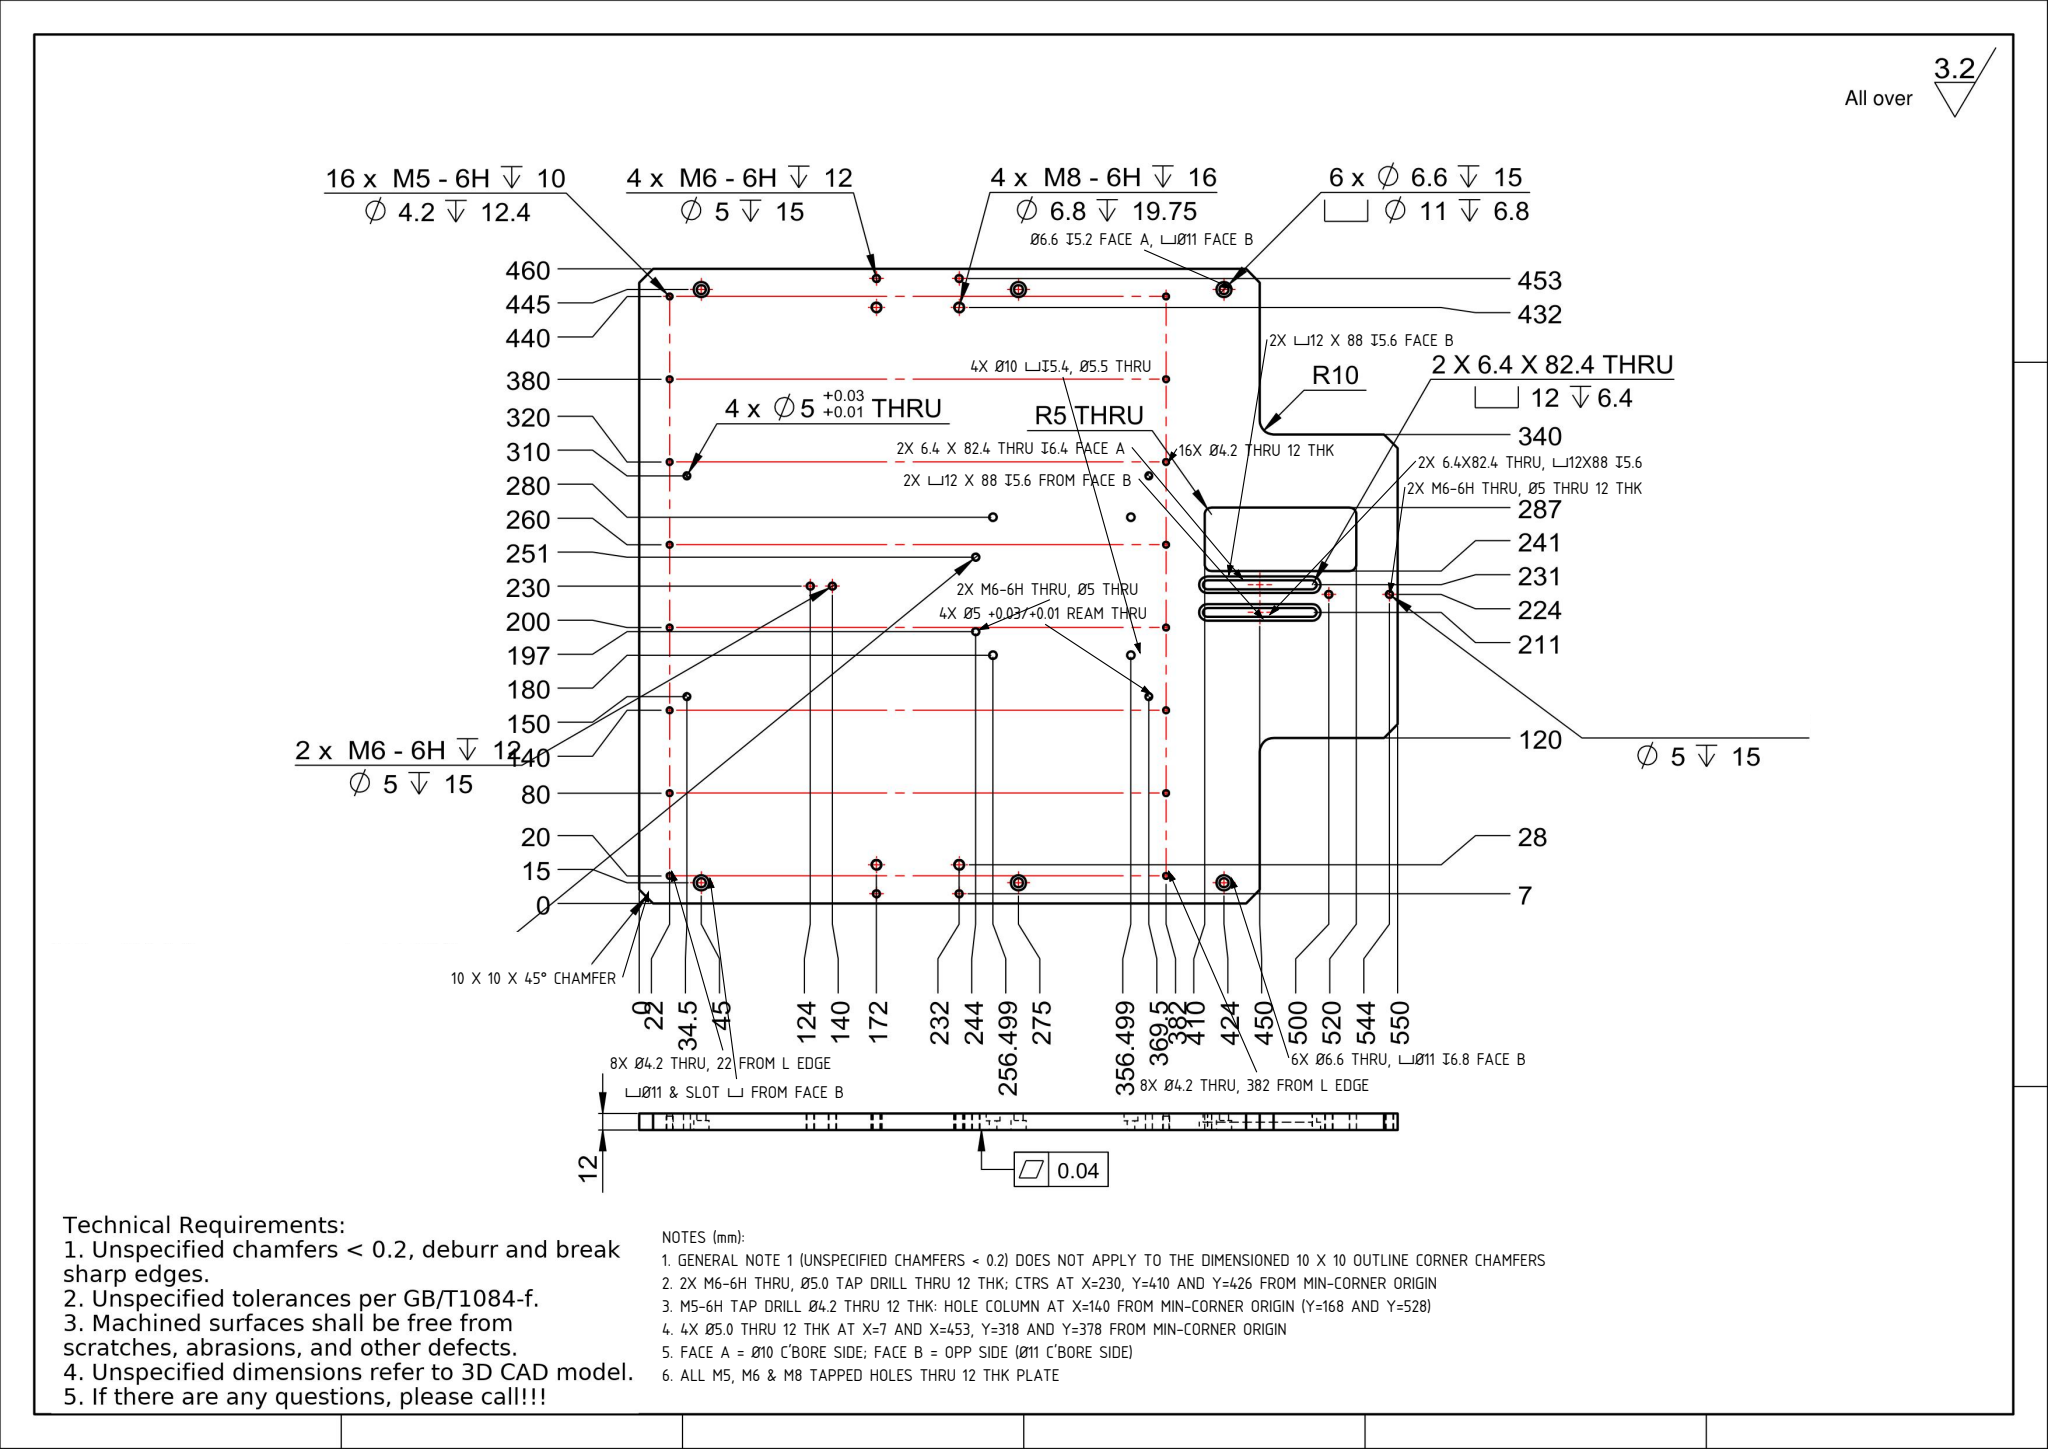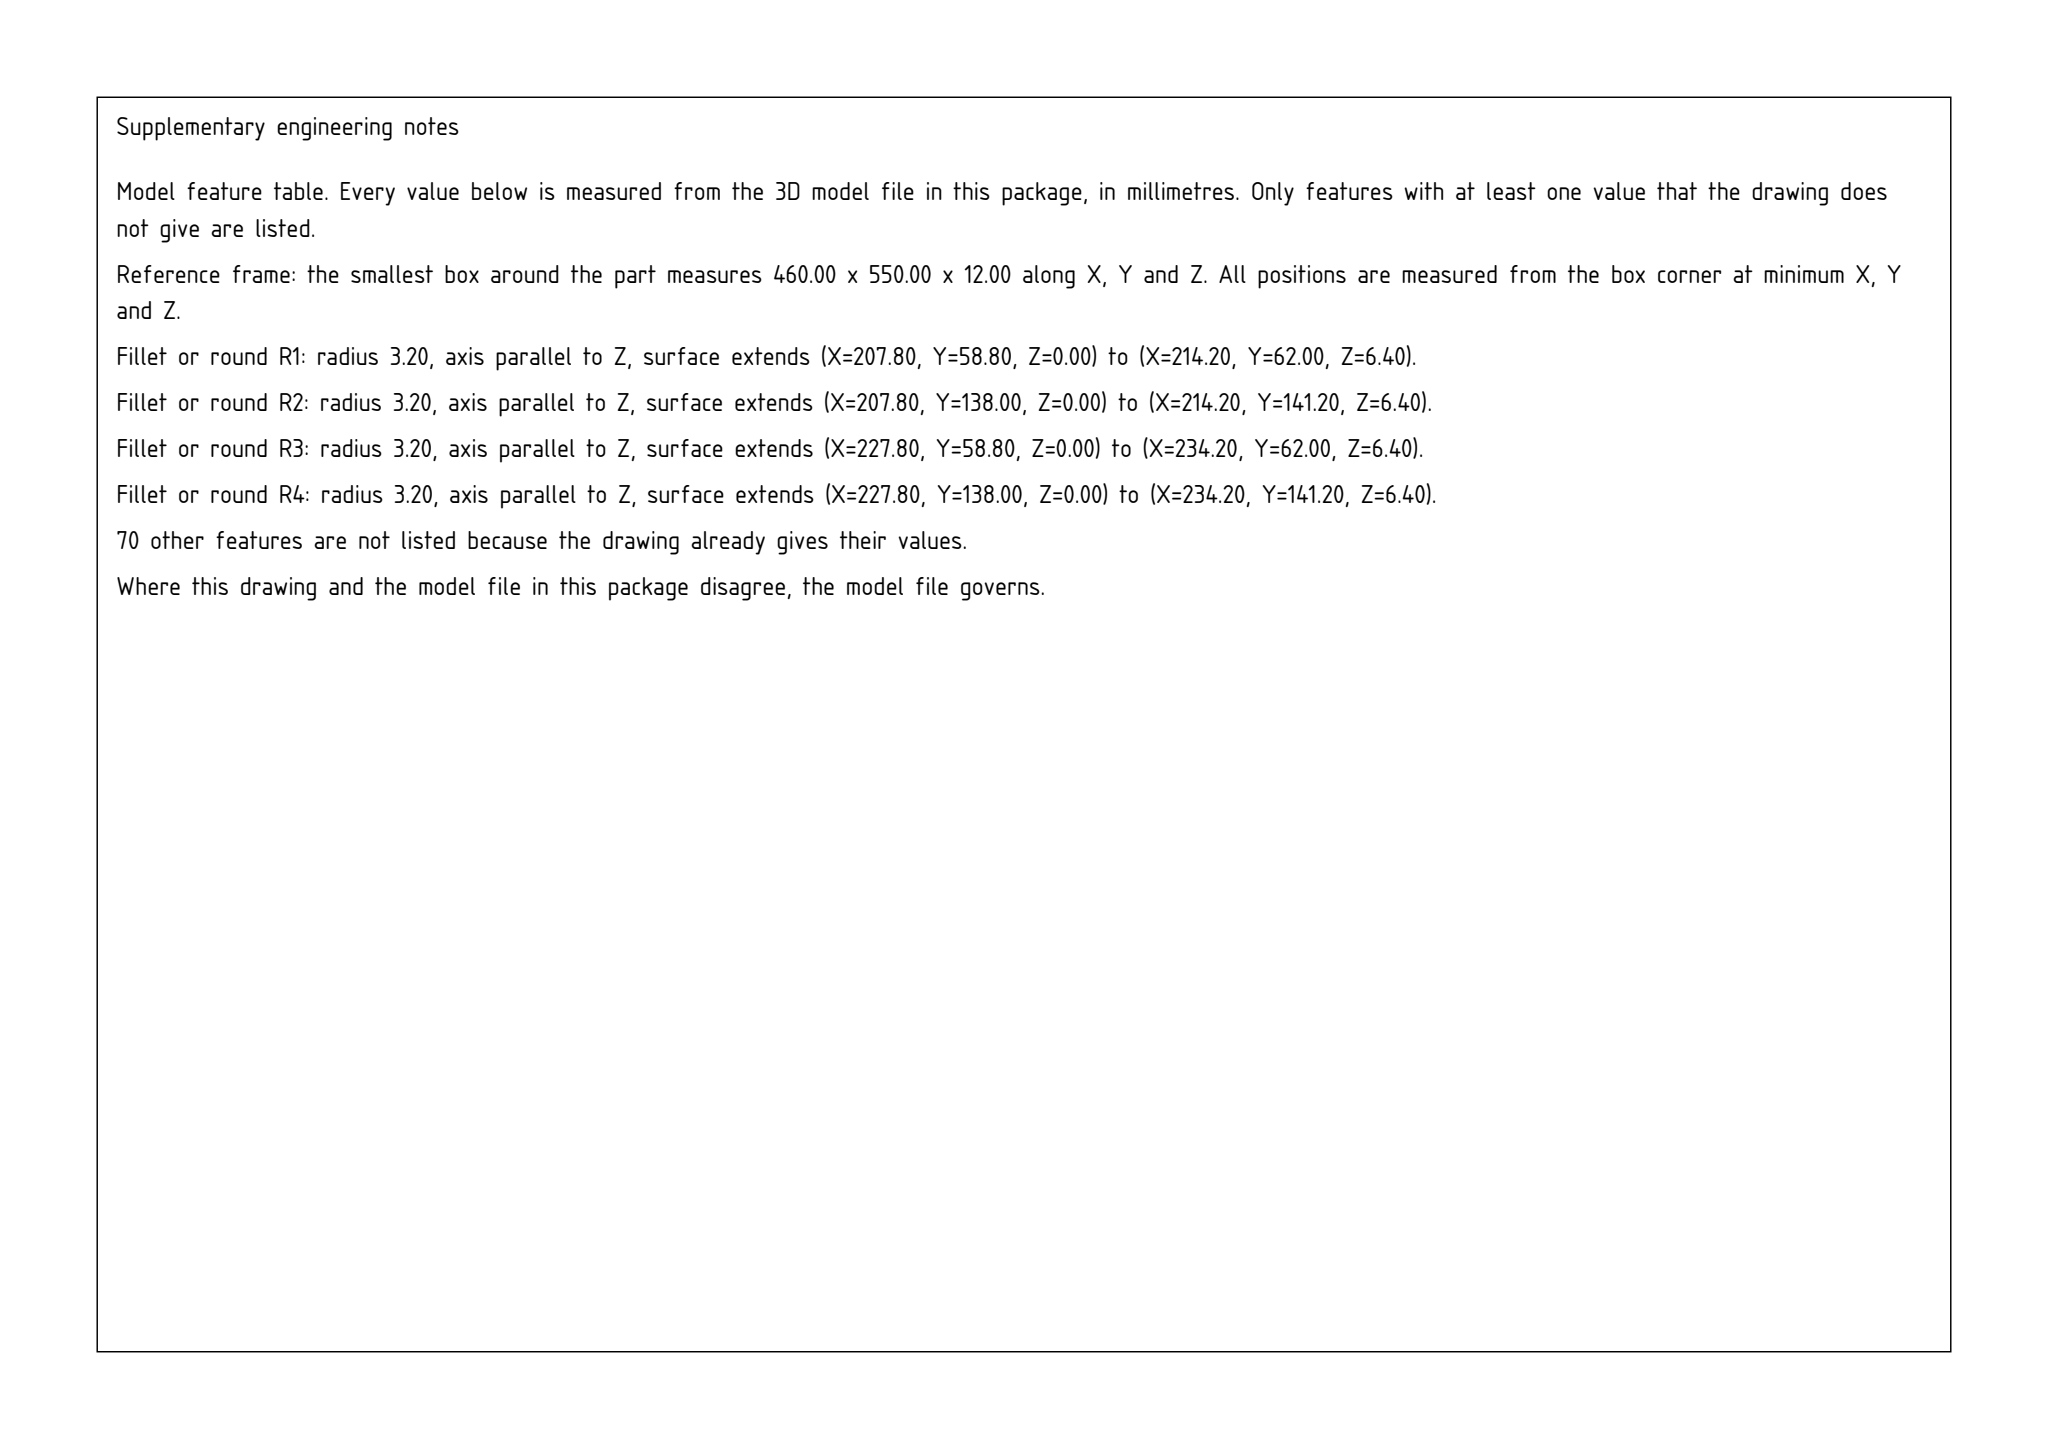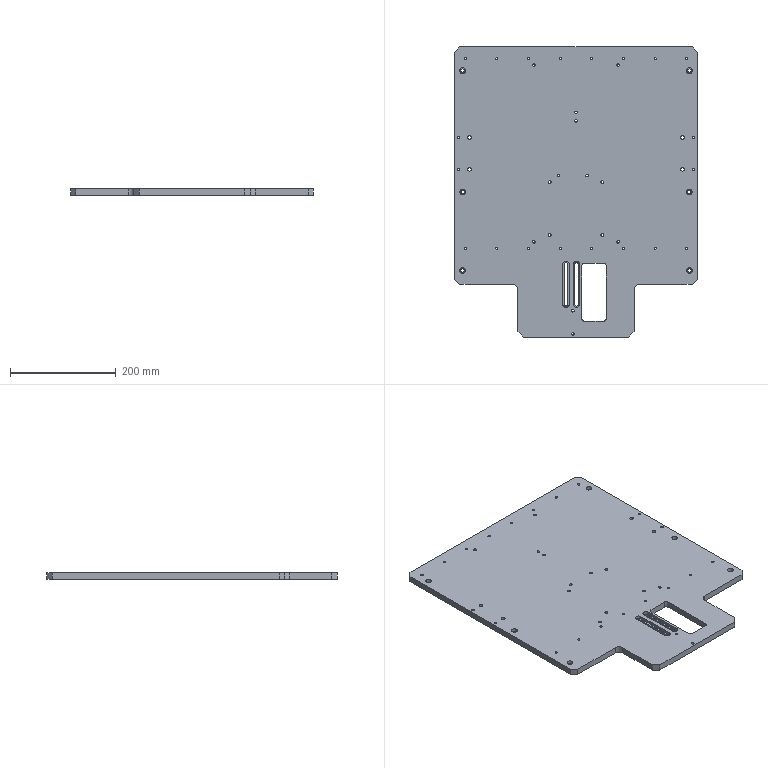Part | SolidWorks | mm | 1 solid | 162 faces | box 460 x 550 x 12 mm | volume 2651363 mm3 | cylinder 122 | plane 40 | commonest cylinder face diameters 4.2 x32 5 x28 10 x12 11 x12 6.6 x12 5.5 x8 6.8 x8 12 x4
Drawing notes:
SLOT C'BORE: 2X C'BORE 12 WIDE X 88 LG (R6 ENDS, END R CTRS AT 412 & 488 FROM LEFT EDGE), DP 5.6 FROM FACE B (OPPOSITE FACE TO THE Ø10 C'BORES), CL AT 211 & 231 FROM BOTTOM EDGE | from the solid: Ø12 slot-end arcs at (211,62),(211,138),(231,62),(231,138) run z 6.4→12 (depth 5.6 from the z=12 face, opposite the Ø10 c'bores at z 0→5.4); the z=6.4 c'bore floor planes extend y 56–144 x 12 wide (205–217 and 225–237), i.e. 88 long with R6 centers at y 62 & 138 = 488 & 412 from left edge (550-y).
SLOT THRU PORTION: 2X 6.4 WIDE X 82.4 LG SLOT (R3.2 ENDS), DP 6.4 FROM FACE A (Ø10 C'BORE FACE), CL AT 211 & 231 FROM BOTTOM EDGE | from the solid: Ø6.4 arcs z 0→6.4 at (211,62/138) & (231,62/138); planes x207.8/214.2 and x227.8/234.2, z 0–6.4
FACE DESIGNATION: 6X Ø6.6 DRILLED FROM FACE A DP 5.2; Ø11 C'BORE DP 6.8 MACHINED FROM FACE B (OPPOSITE FACE); THE 4X Ø10 DP 5.4 C'BORES ARE FROM FACE A | from the solid: Ø6.6 z 0→5.2 and Ø11 z 5.2→12; Ø10 z 0→5.4 with Ø5.5 z 5.4→12
16X Ø4.2 TAP DRILL IS THRU THE FULL 12 THK PLATE (DRILL DP 12.4 CALLOUT = THRU) | from the solid: Ø4.2 holes z 0→12 at 20,80,140,200,260,320,380,440 on y=168 and y=528
10 X 10 X 45° CHAMFER (LEG 10 ON EACH EDGE) AT THE OUTLINE CORNERS, FULL 12 THK; INCL. CORNERS AT VERTICAL 0 / HORIZONTAL 450 AND VERTICAL 0 / HORIZONTAL 10 | from the solid: inclined_planes angle 45/45/90, size 10x10x12, bbox_from (0,100,0) and (0,540,0)
GENERAL NOTE 1 (UNSPECIFIED CHAMFERS < 0.2) DOES NOT APPLY TO THE DIMENSIONED 10 X 10 OUTLINE CORNER CHAMFERS | from the solid: inclined_planes 10x10x12 at 45° on outline corners
2X M6-6H THRU, Ø5.0 TAP DRILL THRU 12 THK; CTRS AT X=230, Y=410 AND Y=426 FROM MIN-CORNER ORIGIN | from the solid: cylinders: hole/bore dia 5.0, axis z, at [230.0,410.0] and [230.0,426.0], from 0.0 to 12.0 (full thickness)
M5-6H TAP DRILL Ø4.2 THRU 12 THK: HOLE COLUMN AT X=140 FROM MIN-CORNER ORIGIN (Y=168 AND Y=528) | from the solid: cylinders: hole/bore dia 4.2, axis z, at [140.0,168.0] and [140.0,528.0], from 0.0 to 12.0
4X Ø5 +0.03/+0.01 REAMED THRU 12 THK; CTRS AT X=150 AND X=310, Y=180.5 AND Y=515.5 FROM MIN-CORNER ORIGIN (180.5 = 369.5 FROM THE Y=550 EDGE) | from the solid: cylinders: hole/bore Ø5.0 axis z at (150,180.5), (310,180.5), (150,515.5), (310,515.5), from 0.0 to 12.0
M5-6H TAP DRILL Ø4.2 THRU 12 THK: HOLE ROW AT Y=168 FROM MIN-CORNER ORIGIN (382 FROM THE Y=550 EDGE); X=20, 80, 140, 200, 260, 320, 380, 440 | from the solid: cylinders: hole/bore Ø4.2 axis z at (20,168), (80,168), (140,168), (200,168), (260,168), (320,168), (380,168), (440,168), from 0.0 to 12.0
M5-6H TAP DRILL Ø4.2 THRU 12 THK: HOLE ROW AT Y=528 FROM MIN-CORNER ORIGIN (22 FROM THE Y=550 EDGE); X=20, 80, 140, 200, 260, 320, 380, 440 | from the solid: cylinders: hole/bore Ø4.2 axis z at y=528.0, x=20/80/140/200/260/320/380/440, from z=0.0 to z=12.0
2X M6-6H THRU, Ø5.0 TAP DRILL THRU FULL 12 THK; CTRS AT X=224, Y=6 AND Y=50 FROM MIN-CORNER ORIGIN | from the solid: cylinders: hole/bore dia 5.0, axis z at [224,6] and [224,50], from 0.0 to 12.0 (full plate THK)
2X M6-6H THRU, Ø5.0 TAP DRILL THRU FULL 12 THK; CTRS AT Y=306, X=197 AND X=251 FROM MIN-CORNER ORIGIN (REPLACES THE OVERLAPPED M6 CALLOUT) | from the solid: cylinders: hole/bore dia 5.0, axis z at [197,306] and [251,306], from 0.0 to 12.0
4X Ø5.0 THRU 12 THK AT X=7 AND X=453, Y=318 AND Y=378 FROM MIN-CORNER ORIGIN | from the solid: cylinders: hole/bore dia 5.0, axis z at [7,318], [7,378], [453,318], [453,378], from 0.0 to 12.0
FACE A = Ø10 C'BORE SIDE; FACE B = OPP SIDE (Ø11 C'BORE SIDE) | from the solid: Ø10 c'bores z=0->5.4 (Face A); Ø11 c'bores z=5.2->12.0 (Face B); plate z 0-12
6X Ø11 C'BORE & 2X SLOT C'BORE MACHINED FROM FACE B | from the solid: Ø11 bores from z=5.2 to 12; slot c'bore planes z=6.4 to 12 (x205-217 & x225-237, y56-144)
4X Ø10 CBORE DP 5.4 (Ø5.5 THRU) FROM FACE A | from the solid: Ø10 z=0->5.4 then Ø5.5 z=5.4->12 at (180/280, 193.5/293.5)
2X SLOT C'BORE: CBORE 12 WIDE X 88 LG DP 5.6 FROM FACE B | from the solid: slot c'bore floor plane z=6.4, top z=12 => 5.6 deep; width x205-217=12, y56-144=88
2X 6.4 X 82.4 THRU; CBORE 12 X 88 DP 5.6 FROM FACE B | from the solid: 6.4 wide slot z=0->6.4 breaks into 12 wide c'bore z=6.4->12; thru slot y62-138 + R3.2 ends = 82.4
ALL M5, M6 & M8 TAPPED HOLES THRU 12 THK PLATE | from the solid: Ø4.2, Ø5, Ø6.8 holes all from z=0.0 to z=12.0
6X Ø6.6 THRU, CBORE Ø11 DP 6.8 FROM FACE B | from the solid: Ø6.6 z=0->5.2 + Ø11 z=5.2->12 (6.8 deep) at x15/445, y126/275/505
build123d program:
from build123d import *

# Parameters (mm, degrees)
SKETCH1_W                                         = 460
SKETCH1_H                                         = 550
BOSS_EXTRUDE1_DEPTH                               = 12
SKETCH2_W                                         = 120
SKETCH2_H                                         = 100
CUT_EXTRUDE1_DEPTH                                = 12
FILLET1_R                                         = 10
CHAMFER1_SIZE                                     = 10
SKETCH3_W                                         = 46
SKETCH3_H                                         = 110
CUT_EXTRUDE2_DEPTH                                = 359.705
FILLET2_R                                         = 5
CUT_EXTRUDE3_DEPTH                                = 5.6
CUT_EXTRUDE4_DEPTH                                = 359.561
M6_TAPPED_HOLE1_D                                 = 5
M6_TAPPED_HOLE1_DEPTH                             = 15
M6_TAPPED_HOLE1_TIP                               = 1.502
LPATTERN1_COUNT                                   = 8
LPATTERN1_PITCH                                   = 60
LPATTERN1_COUNT_DIR2                              = 2
LPATTERN1_PITCH_DIR2                              = 360
M6_TAPPED_HOLE2_D                                 = 5
M6_TAPPED_HOLE2_DEPTH                             = 15
M6_TAPPED_HOLE2_TIP                               = 1.502
M8_TAPPED_HOLE1_D                                 = 6.8
M8_TAPPED_HOLE1_DEPTH                             = 19.75
M8_TAPPED_HOLE1_TIP                               = 2.043
M6_TAPPED_HOLE3_AT_2_COUNT                        = 2
M6_TAPPED_HOLE3_AT_2_PITCH                        = 60
HOLE_SIZE_ACCORDING_TO_HEXAGON_SOCKET_D           = 6.6
HOLE_SIZE_ACCORDING_TO_HEXAGON_SOCKET_DEPTH       = 15
HOLE_SIZE_ACCORDING_TO_HEXAGON_SOCKET_CBORE_D     = 11
HOLE_SIZE_ACCORDING_TO_HEXAGON_SOCKET_CBORE_DEPTH = 6.8
HOLE_SIZE_ACCORDING_TO_HEXAGON_SOCKET_TIP         = 1.983
SIZE_MM_DOWEL_PIN_HOLE1_D                         = 5
M5_HEX_SOCKET_HEAD_CAP_SCREW_CBORE1_D             = 5.5
M5_HEX_SOCKET_HEAD_CAP_SCREW_CBORE1_DEPTH         = 12.4
M5_HEX_SOCKET_HEAD_CAP_SCREW_CBORE1_CBORE_D       = 10
M5_HEX_SOCKET_HEAD_CAP_SCREW_CBORE1_CBORE_DEPTH   = 5.4
M5_HEX_SOCKET_HEAD_CAP_SCREW_CBORE1_TIP           = 1.652
M6_TAPPED_HOLE4_D                                 = 5


with BuildPart() as part:
    # Sketch1 → Boss-Extrude1 (new body)
    with BuildSketch(Plane.XY):
        Rectangle(SKETCH1_W, SKETCH1_H)
    extrude(amount=BOSS_EXTRUDE1_DEPTH)

    # Sketch2 → Cut-Extrude1 (cut)
    with BuildSketch(Plane.XY.offset(12)):
        with Locations((-170, -225)):
            Rectangle(SKETCH2_W, SKETCH2_H)
        with Locations((170, -225)):
            Rectangle(SKETCH2_W, SKETCH2_H)
    extrude(amount=-CUT_EXTRUDE1_DEPTH, mode=Mode.SUBTRACT)

    # Fillet1
    fillet1_edges = [part.edges().sort_by_distance(p)[0] for p in [
        (-110, -175, 6),
        (110, -175, 6),
    ]]
    fillet(fillet1_edges, radius=FILLET1_R)

    # Chamfer1
    chamfer1_edges = [part.edges().sort_by_distance(p)[0] for p in [
        (-230, -175, 6),
        (-110, -275, 6),
        (110, -275, 6),
        (230, -175, 6),
        (-230, 275, 6),
        (230, 275, 6),
    ]]
    chamfer(chamfer1_edges, length=CHAMFER1_SIZE)

    # Sketch3 → Cut-Extrude2 (cut, through all)
    with BuildSketch(Plane.XY.offset(12)):
        with Locations((34, -190)):
            Rectangle(SKETCH3_W, SKETCH3_H)
    extrude(amount=-CUT_EXTRUDE2_DEPTH, mode=Mode.SUBTRACT)

    # Fillet2
    fillet2_edges = [part.edges().sort_by_distance(p)[0] for p in [
        (57, -135, 6),
        (57, -245, 6),
        (11, -245, 6),
        (11, -135, 6),
    ]]
    fillet(fillet2_edges, radius=FILLET2_R)

    # Sketch4 → Cut-Extrude3 (cut)
    with BuildSketch(Plane.XY.offset(12)):
        with BuildLine():
            Line((7, -137), (7, -213))
            ThreePointArc((7, -213), (1, -219), (-5, -213))
            Line((-5, -213), (-5, -137))
            ThreePointArc((-5, -137), (1, -131), (7, -137))
        make_face()
        with BuildLine():
            Line((-13, -137), (-13, -213))
            ThreePointArc((-13, -213), (-19, -219), (-25, -213))
            Line((-25, -213), (-25, -137))
            ThreePointArc((-25, -137), (-19, -131), (-13, -137))
        make_face()
    extrude(amount=-CUT_EXTRUDE3_DEPTH, mode=Mode.SUBTRACT)

    # Sketch5 → Cut-Extrude4 (cut, through all)
    with BuildSketch(Plane.XY.offset(6.4)):
        with BuildLine():
            Line((4.2, -137), (4.2, -213))
            ThreePointArc((4.2, -213), (1, -216.2), (-2.2, -213))
            Line((-2.2, -213), (-2.2, -137))
            ThreePointArc((-2.2, -137), (1, -133.8), (4.2, -137))
        make_face()
        with BuildLine():
            Line((-15.8, -137), (-15.8, -213))
            ThreePointArc((-15.8, -213), (-19, -216.2), (-22.2, -213))
            Line((-22.2, -213), (-22.2, -137))
            ThreePointArc((-22.2, -137), (-19, -133.8), (-15.8, -137))
        make_face()
    extrude(amount=-CUT_EXTRUDE4_DEPTH, mode=Mode.SUBTRACT)

    # M6 Tapped Hole1
    with Locations(Plane.XY.offset(12)):
        with Locations((-6, -269), (-6, -225)):
            Hole(M6_TAPPED_HOLE1_D / 2, depth=M6_TAPPED_HOLE1_DEPTH)
            with Locations((0, 0, -(M6_TAPPED_HOLE1_DEPTH + M6_TAPPED_HOLE1_TIP / 2))):  # 118° drill point
                Cone(0, M6_TAPPED_HOLE1_D / 2, M6_TAPPED_HOLE1_TIP, mode=Mode.SUBTRACT)

    # Sketch9 → M5 Tapped Hole1 (revolve, cut)
    with BuildSketch(Plane(origin=(-210, -107, 12), x_dir=(0, -1, 0), z_dir=(1, 0, 0))):
        Polygon((0, 0), (0, 13.662), (2.1, 12.4), (2.1, 0), align=None)
    m5_tapped_hole1 = revolve(axis=Axis((-210, -107, 18.35), (0, 0, -1)), mode=Mode.SUBTRACT)

    # LPattern1: M5 Tapped Hole1 8 × 2
    with Locations(*[(i * LPATTERN1_PITCH, j * LPATTERN1_PITCH_DIR2, 0) for i in range(LPATTERN1_COUNT) for j in range(LPATTERN1_COUNT_DIR2) if (i, j) != (0, 0)]):
        add(m5_tapped_hole1, mode=Mode.SUBTRACT)

    # M6 Tapped Hole2
    with Locations(Plane.XY.offset(12)):
        with Locations((0, 151), (0, 135)):
            Hole(M6_TAPPED_HOLE2_D / 2, depth=M6_TAPPED_HOLE2_DEPTH)
            with Locations((0, 0, -(M6_TAPPED_HOLE2_DEPTH + M6_TAPPED_HOLE2_TIP / 2))):  # 118° drill point
                Cone(0, M6_TAPPED_HOLE2_D / 2, M6_TAPPED_HOLE2_TIP, mode=Mode.SUBTRACT)

    # M8 Tapped Hole1
    with Locations(Plane.XY.offset(12)):
        with Locations((202, 103), (202, 43), (-202, 103), (-202, 43)):
            Hole(M8_TAPPED_HOLE1_D / 2, depth=M8_TAPPED_HOLE1_DEPTH)
            with Locations((0, 0, -(M8_TAPPED_HOLE1_DEPTH + M8_TAPPED_HOLE1_TIP / 2))):  # 118° drill point
                Cone(0, M8_TAPPED_HOLE1_D / 2, M8_TAPPED_HOLE1_TIP, mode=Mode.SUBTRACT)

    # Sketch16 → M6 Tapped Hole3 (revolve, cut)
    with BuildSketch(Plane(origin=(223, 103, 12), x_dir=(0, -1, 0), z_dir=(1, 0, 0))):
        Polygon((0, 0), (0, 16.502), (2.5, 15), (2.5, 0), align=None)
    m6_tapped_hole3 = revolve(axis=Axis((223, 103, 18.35), (0, 0, -1)), mode=Mode.SUBTRACT)

    # M6 Tapped Hole3 at 2: M6 Tapped Hole3 ×2
    with Locations(*[(0, -i * M6_TAPPED_HOLE3_AT_2_PITCH, 0) for i in range(1, M6_TAPPED_HOLE3_AT_2_COUNT)]):
        add(m6_tapped_hole3, mode=Mode.SUBTRACT)

    # Hole Size _ according to_ Hexagon Socket
    with Locations(Plane.XY.offset(12)):
        with Locations((-215, 230), (-215, 0), (-215, -149), (215, -149), (215, 0), (215, 230)):
            CounterBoreHole(HOLE_SIZE_ACCORDING_TO_HEXAGON_SOCKET_D / 2, HOLE_SIZE_ACCORDING_TO_HEXAGON_SOCKET_CBORE_D / 2, HOLE_SIZE_ACCORDING_TO_HEXAGON_SOCKET_CBORE_DEPTH, depth=HOLE_SIZE_ACCORDING_TO_HEXAGON_SOCKET_DEPTH)
            with Locations((0, 0, -(HOLE_SIZE_ACCORDING_TO_HEXAGON_SOCKET_DEPTH + HOLE_SIZE_ACCORDING_TO_HEXAGON_SOCKET_TIP / 2))):  # 118° drill point
                Cone(0, HOLE_SIZE_ACCORDING_TO_HEXAGON_SOCKET_D / 2, HOLE_SIZE_ACCORDING_TO_HEXAGON_SOCKET_TIP, mode=Mode.SUBTRACT)

    # Size mm Dowel Pin Hole1 (through all)
    with Locations(Plane.XY.offset(12)):
        with Locations((-80, -94.5), (80, -94.5), (-80, 240.5), (80, 240.5)):
            Hole(SIZE_MM_DOWEL_PIN_HOLE1_D / 2)

    # Mirror1: M6 Tapped Hole3 across plane
    add(m6_tapped_hole3.mirror(Plane(origin=(0, 0, 0), x_dir=(0, 0, 1), z_dir=(1, 0, 0))), mode=Mode.SUBTRACT)

    # Mirror1 copy 1 sketch → Mirror1 copy 1 (revolve, cut)
    with BuildSketch(Plane(origin=(-223, 43, 12), x_dir=(0, -1, 0), z_dir=(-1, 0, 0))):
        Polygon((0, 0), (0, -16.502), (2.5, -15), (2.5, 0), align=None)
    revolve(axis=Axis((-223, 43, 18.35), (0, 0, 1)), mode=Mode.SUBTRACT)

    # M5 Hex Socket Head Cap Screw CBORE1
    with Locations(Plane(origin=(0, 0, 0), x_dir=(-1, 0, 0), z_dir=(0, 0, -1))):
        with Locations((50, 18.501), (-50, 18.501), (-50, -81.499), (50, -81.499)):
            CounterBoreHole(M5_HEX_SOCKET_HEAD_CAP_SCREW_CBORE1_D / 2, M5_HEX_SOCKET_HEAD_CAP_SCREW_CBORE1_CBORE_D / 2, M5_HEX_SOCKET_HEAD_CAP_SCREW_CBORE1_CBORE_DEPTH, depth=M5_HEX_SOCKET_HEAD_CAP_SCREW_CBORE1_DEPTH)
            with Locations((0, 0, -(M5_HEX_SOCKET_HEAD_CAP_SCREW_CBORE1_DEPTH + M5_HEX_SOCKET_HEAD_CAP_SCREW_CBORE1_TIP / 2))):  # 118° drill point
                Cone(0, M5_HEX_SOCKET_HEAD_CAP_SCREW_CBORE1_D / 2, M5_HEX_SOCKET_HEAD_CAP_SCREW_CBORE1_TIP, mode=Mode.SUBTRACT)

    # M6 Tapped Hole4 (through all)
    with Locations(Plane.XY.offset(12)):
        with Locations((21, 31), (-33, 31)):
            Hole(M6_TAPPED_HOLE4_D / 2)


solid = part.part